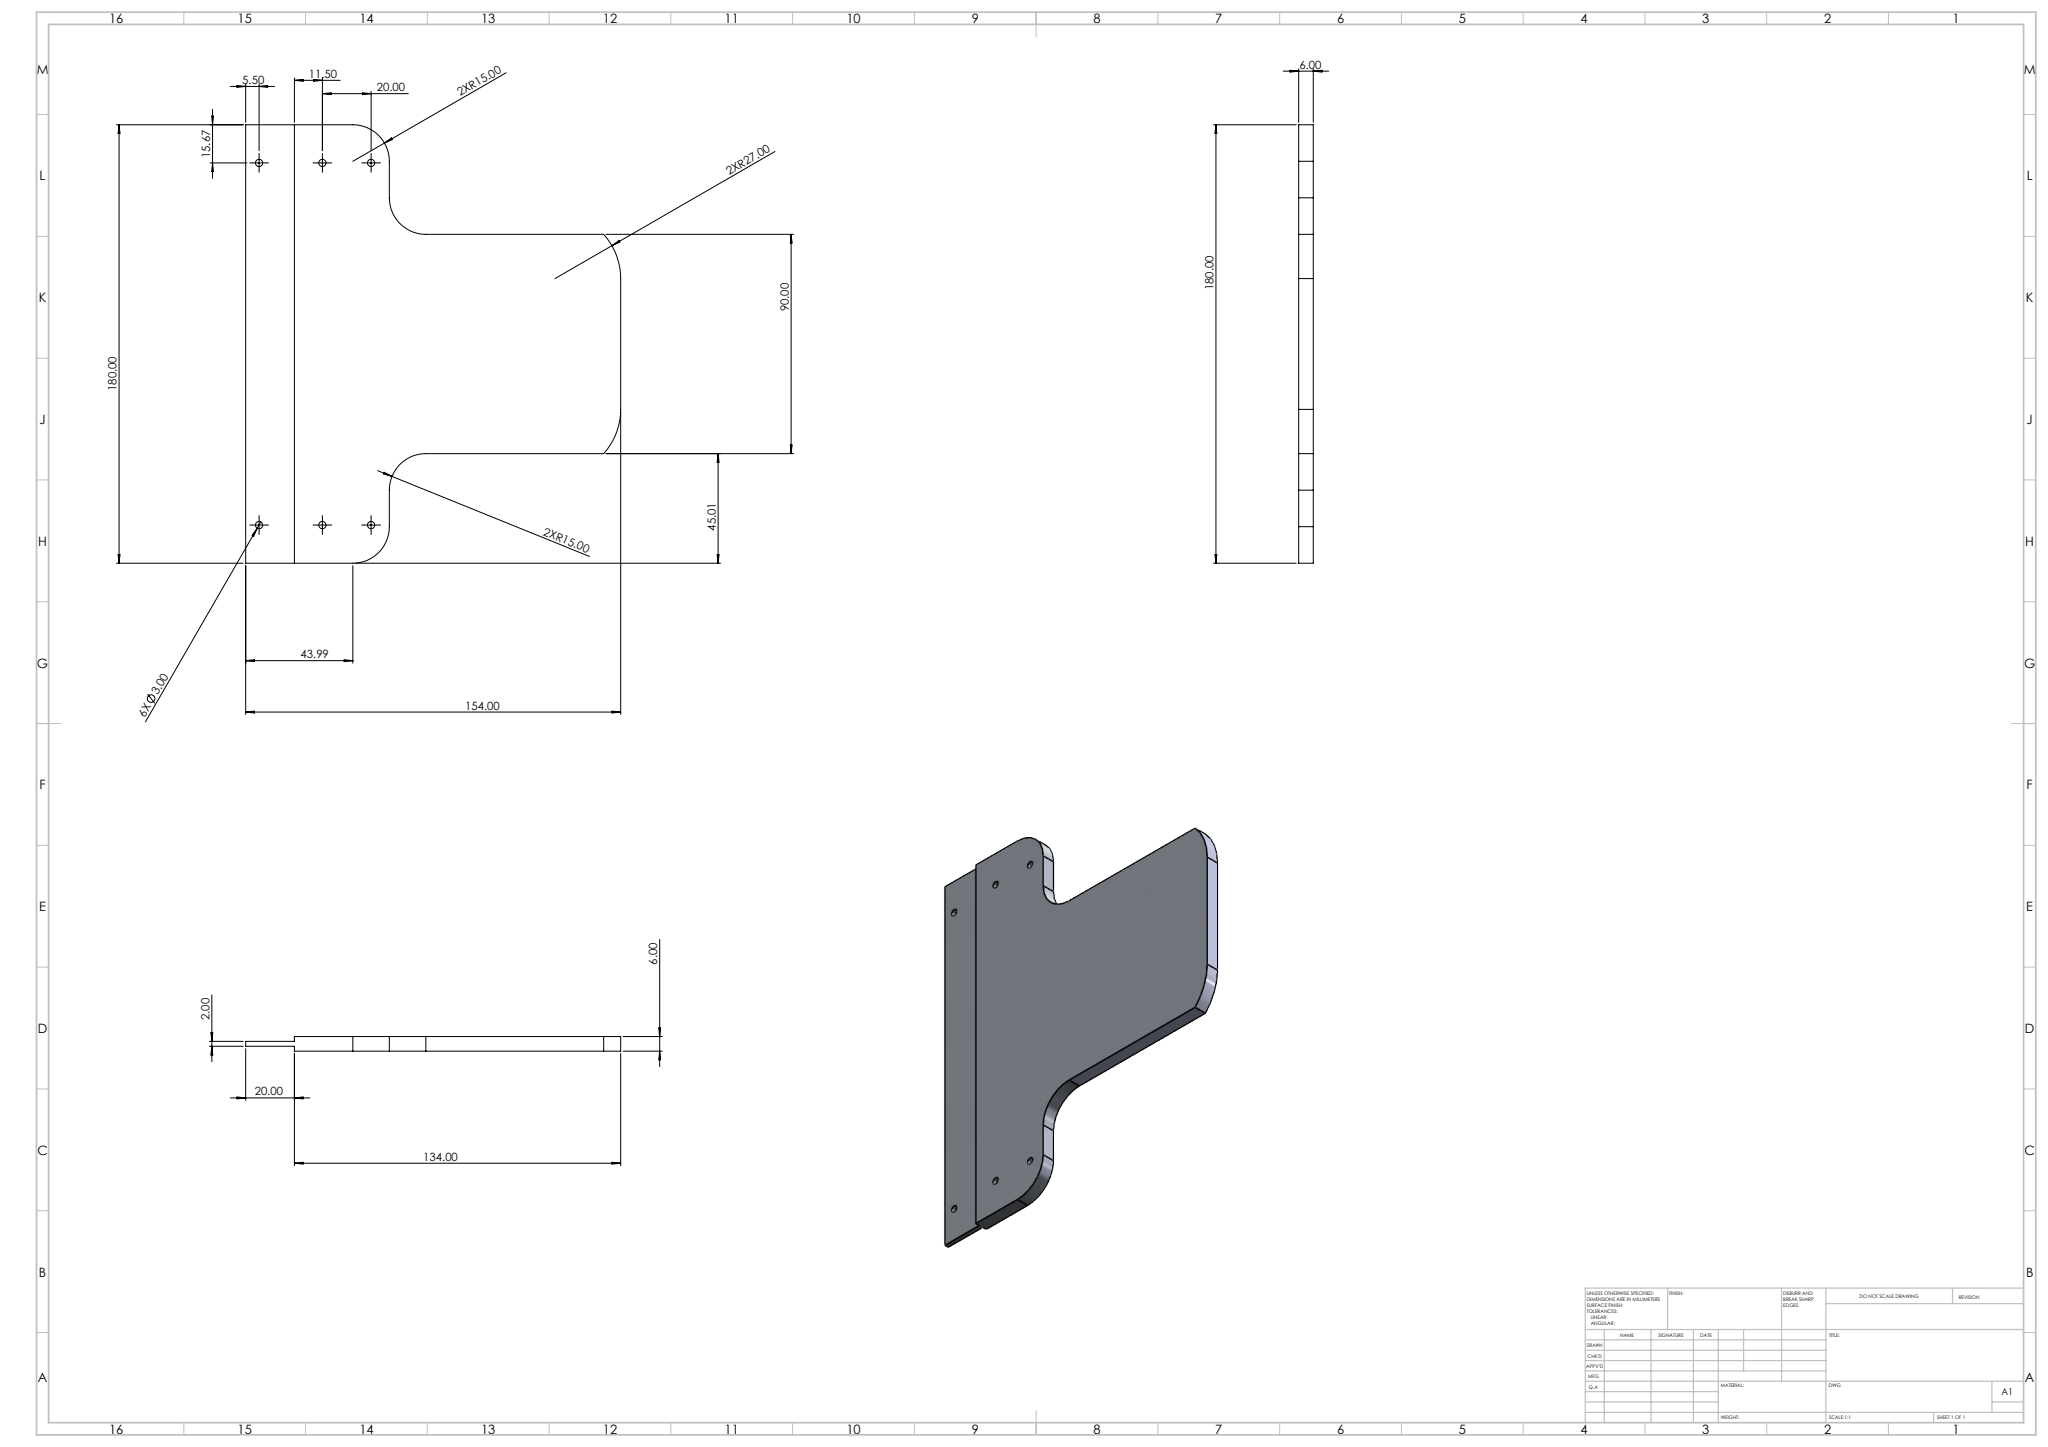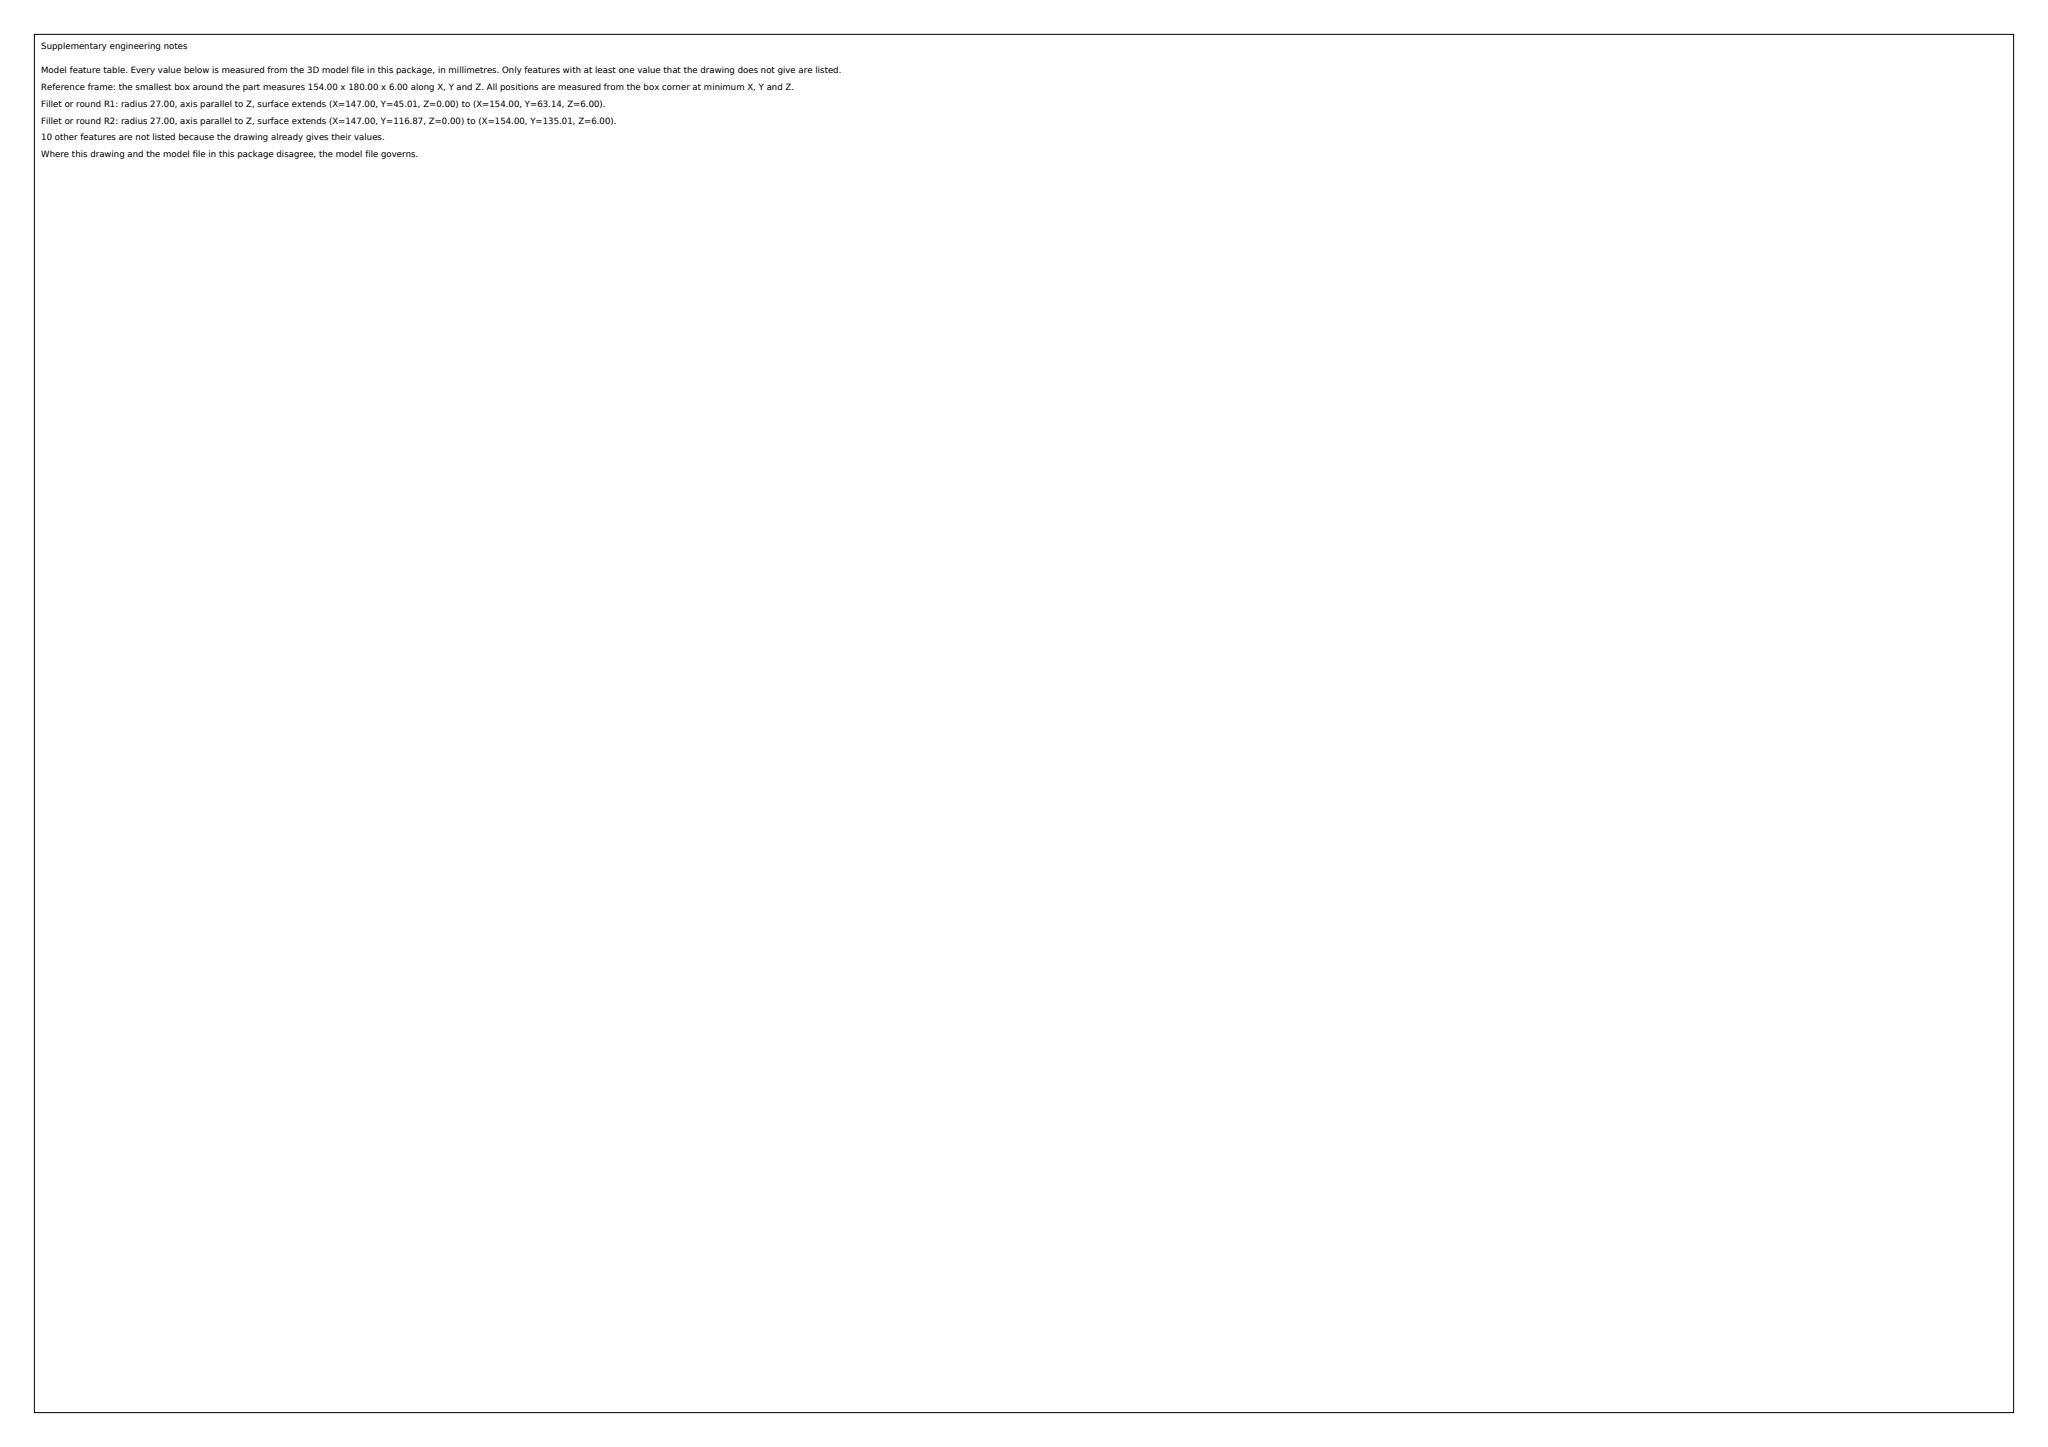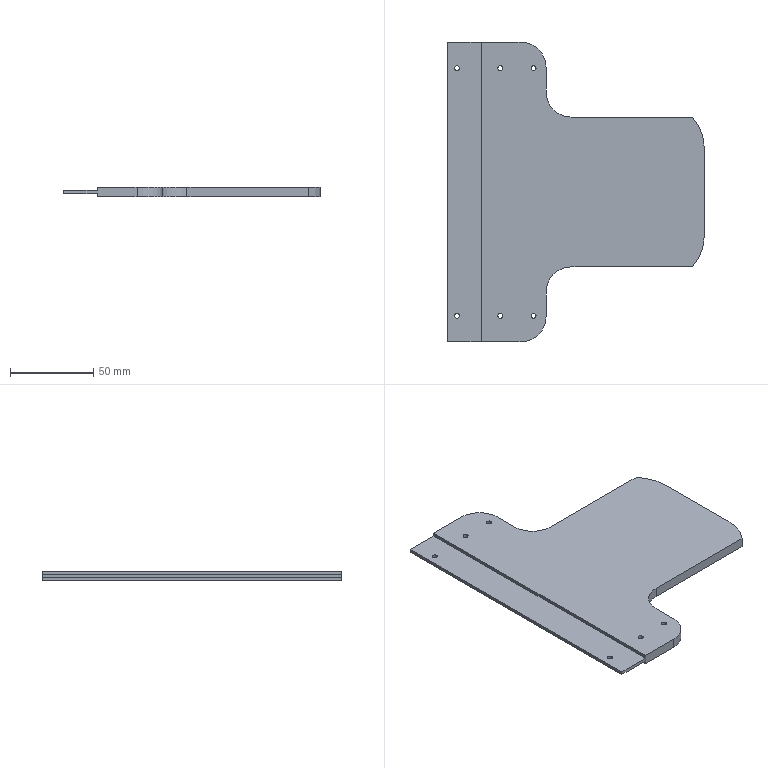Part | SolidWorks | mm | 1 solid | 33 faces | box 154 x 180 x 6 mm | volume 99941 mm3 | cylinder 19 | plane 14 | commonest cylinder face diameters 3 x12 30 x5 54 x2
build123d program:
from build123d import *

# Parameters (mm, degrees)
BOSS_EXTRUDE1_DEPTH = 6
SKETCH3_W           = 2
SKETCH3_H           = 180
BOSS_EXTRUDE2_DEPTH = 20
SKETCH7_R           = 1.5
CUT_EXTRUDE2_DEPTH  = 10


with BuildPart() as part:
    # Sketch2 → Boss-Extrude1 (new body)
    with BuildSketch(Plane.XY):
        with BuildLine():
            Line((-7.653, 45), (-29.666, 45))
            ThreePointArc((-29.666, 45), (-40.273, 49.393), (-44.666, 60))
            Line((-44.666, 60), (-44.666, 74.994))
            ThreePointArc((-44.666, 74.994), (-49.059, 85.6), (-59.666, 89.994))
            Line((-59.666, 89.994), (-83.666, 89.994))
            Line((-83.666, 89.994), (-83.666, -90.006))
            Line((-83.666, -90.006), (-59.672, -90.006))
            ThreePointArc((-59.672, -90.006), (-49.064, -85.611), (-44.672, -75))
            Line((-44.672, -75), (-44.679, -60.006))
            ThreePointArc((-44.679, -60.006), (-40.288, -49.396), (-29.679, -45))
            Line((-29.679, -45), (-7.666, -45))
            Line((-7.666, -45), (18.334, -45))
            Line((18.334, -45), (43.334, -45))
            ThreePointArc((43.334, -45), (48.523, -36.583), (50.334, -26.862))
            Line((50.334, -26.862), (50.334, 26.862))
            ThreePointArc((50.334, 26.862), (48.523, 36.583), (43.334, 45))
            Line((43.334, 45), (18.334, 45))
            Line((18.334, 45), (-7.653, 45))
        make_face()
    extrude(amount=BOSS_EXTRUDE1_DEPTH)

    # Sketch3 → Boss-Extrude2 (add)
    with BuildSketch(Plane.ZY.offset(83.666)):
        with Locations((3, -0.006497)):
            Rectangle(SKETCH3_W, SKETCH3_H)
    extrude(amount=BOSS_EXTRUDE2_DEPTH)

    # Sketch7 → Cut-Extrude2 (cut)
    with BuildSketch(Plane(origin=(0, 0, 0), x_dir=(-1, 0, 0), z_dir=(0, 0, -1))):
        with Locations((52.173, -74.336)):
            Circle(SKETCH7_R)
        with Locations(Location((52.166, 74.324, 0), (0, 0, 180))):
            Circle(SKETCH7_R)
        with Locations((72.173, -74.336)):
            Circle(SKETCH7_R)
        with Locations((72.166, 74.324)):
            Circle(SKETCH7_R)
        with Locations(Location((98.166, -74.336, 0), (0, 0, 90))):
            Circle(SKETCH7_R)
        with Locations(Location((98.166, 74.324, 0), (0, 0, 90))):
            Circle(SKETCH7_R)
    extrude(amount=-CUT_EXTRUDE2_DEPTH, mode=Mode.SUBTRACT)


solid = part.part